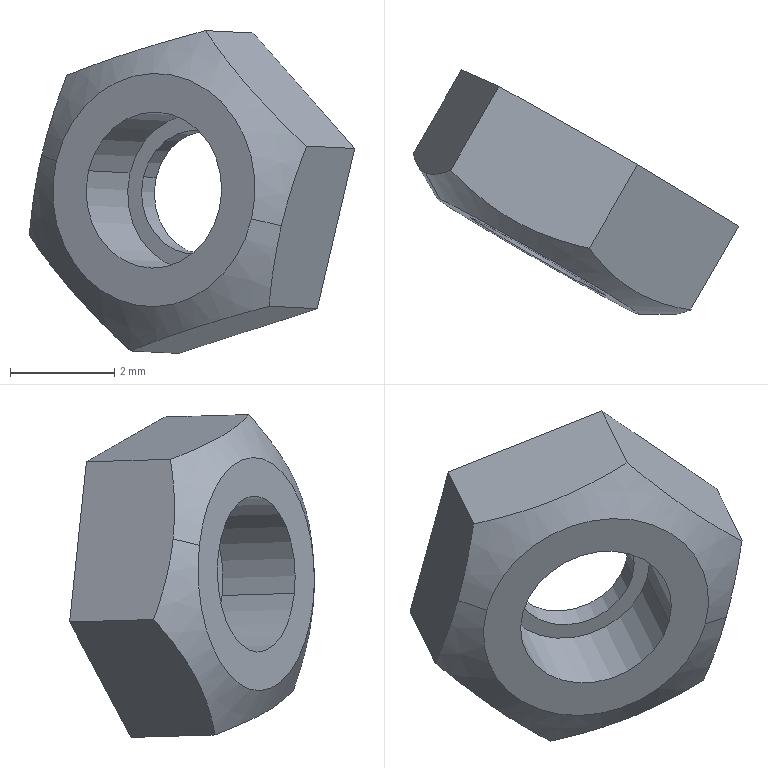Component | SolidWorks | KKSwitch-0710z0-123-1_CBTN3-0710z0-123-11 | 1 solid | 17 faces | box 6.25 x 4.7 x 6.2 mm | volume 45 mm3 | plane 9 | cylinder 4 | cone 4 | commonest cylinder face diameters 3 x2 2.386 x2
STEP:
#1=COLOUR_RGB('',0.7922,0.8196,0.9333);
#2=FILL_AREA_STYLE_COLOUR('',#1);
#3=FILL_AREA_STYLE('',(#2));
#4=SURFACE_STYLE_FILL_AREA(#3);
#5=SURFACE_SIDE_STYLE('',(#4));
#6=SURFACE_STYLE_USAGE(.BOTH.,#5);
#7=PRESENTATION_STYLE_ASSIGNMENT((#6));
#8=CARTESIAN_POINT('',(2.602,-0.2727,9.583));
#9=VERTEX_POINT('',#8);
#10=CARTESIAN_POINT('',(2.503,-0.2151,9.612));
#11=VERTEX_POINT('',#10);
#12=CARTESIAN_POINT('',(2.553,-0.2439,9.598));
#13=DIRECTION('',(-0.4977,-0.867,0.02519));
#14=DIRECTION('',(-0.8373,0.4878,0.2469));
#15=AXIS2_PLACEMENT_3D('',#12,#13,#14);
#16=CIRCLE('',#15,0.05906);
#17=EDGE_CURVE('',#9,#11,#16,.T.);
#18=ORIENTED_EDGE('',*,*,#17,.F.);
#19=CARTESIAN_POINT('',(2.571,-0.3273,9.585));
#20=VERTEX_POINT('',#19);
#21=CARTESIAN_POINT('',(2.54,-0.382,9.586));
#22=DIRECTION('',(-0.4977,-0.867,0.02519));
#23=VECTOR('',#22,39.37);
#24=LINE('',#21,#23);
#25=EDGE_CURVE('',#9,#20,#24,.T.);
#26=ORIENTED_EDGE('',*,*,#25,.T.);
#27=CARTESIAN_POINT('',(2.472,-0.2697,9.614));
#28=VERTEX_POINT('',#27);
#29=CARTESIAN_POINT('',(2.522,-0.2985,9.599));
#30=DIRECTION('',(-0.4977,-0.867,0.02519));
#31=DIRECTION('',(-0.8373,0.4878,0.2469));
#32=AXIS2_PLACEMENT_3D('',#29,#30,#31);
#33=CIRCLE('',#32,0.05906);
#34=EDGE_CURVE('',#20,#28,#33,.T.);
#35=ORIENTED_EDGE('',*,*,#34,.T.);
#36=CARTESIAN_POINT('',(2.441,-0.3243,9.615));
#37=DIRECTION('',(-0.4977,-0.867,0.02519));
#38=VECTOR('',#37,39.37);
#39=LINE('',#36,#38);
#40=EDGE_CURVE('',#11,#28,#39,.T.);
#41=ORIENTED_EDGE('',*,*,#40,.F.);
#42=EDGE_LOOP('',(#18,#26,#35,#41));
#43=FACE_OUTER_BOUND('',#42,.T.);
#44=CARTESIAN_POINT('',(2.49,-0.3531,9.601));
#45=DIRECTION('',(-0.4977,-0.867,0.02519));
#46=DIRECTION('',(-0.8373,0.4878,0.2469));
#47=AXIS2_PLACEMENT_3D('',#44,#45,#46);
#48=CYLINDRICAL_SURFACE('',#47,0.05906);
#49=ADVANCED_FACE('',(#43),#48,.F.);
#50=CARTESIAN_POINT('',(2.523,-0.2042,9.609));
#51=VERTEX_POINT('',#50);
#52=CARTESIAN_POINT('',(2.602,-0.25,9.586));
#53=VERTEX_POINT('',#52);
#54=CARTESIAN_POINT('',(2.563,-0.2271,9.597));
#55=DIRECTION('',(0.4977,0.867,-0.02519));
#56=DIRECTION('',(-0.2264,0.1018,-0.9687));
#57=AXIS2_PLACEMENT_3D('',#54,#55,#56);
#58=CIRCLE('',#57,0.04696);
#59=EDGE_CURVE('',#51,#53,#58,.T.);
#60=ORIENTED_EDGE('',*,*,#59,.F.);
#61=CARTESIAN_POINT('',(2.519,-0.1878,9.611));
#62=VERTEX_POINT('',#61);
#63=CARTESIAN_POINT('',(2.519,-0.1878,9.611));
#64=DIRECTION('',(-0.2401,0.958,0.1568));
#65=VECTOR('',#64,39.37);
#66=LINE('',#63,#65);
#67=EDGE_CURVE('',#51,#62,#66,.T.);
#68=ORIENTED_EDGE('',*,*,#67,.T.);
#69=CARTESIAN_POINT('',(2.618,-0.2454,9.582));
#70=VERTEX_POINT('',#69);
#71=CARTESIAN_POINT('',(2.569,-0.2166,9.597));
#72=DIRECTION('',(-0.4977,-0.867,0.02519));
#73=DIRECTION('',(0.8373,-0.4878,-0.2469));
#74=AXIS2_PLACEMENT_3D('',#71,#72,#73);
#75=CIRCLE('',#74,0.05906);
#76=EDGE_CURVE('',#70,#62,#75,.T.);
#77=ORIENTED_EDGE('',*,*,#76,.F.);
#78=CARTESIAN_POINT('',(2.618,-0.2454,9.582));
#79=DIRECTION('',(0.944,0.2681,-0.1924));
#80=VECTOR('',#79,39.37);
#81=LINE('',#78,#80);
#82=EDGE_CURVE('',#53,#70,#81,.T.);
#83=ORIENTED_EDGE('',*,*,#82,.F.);
#84=EDGE_LOOP('',(#60,#68,#77,#83));
#85=FACE_OUTER_BOUND('',#84,.T.);
#86=CARTESIAN_POINT('',(2.569,-0.2166,9.597));
#87=DIRECTION('',(0.4977,0.867,-0.02519));
#88=DIRECTION('',(0.8373,-0.4878,-0.2469));
#89=AXIS2_PLACEMENT_3D('',#86,#87,#88);
#90=CONICAL_SURFACE('',#89,0.05906,0.7854);
#91=ADVANCED_FACE('',(#85),#90,.F.);
#92=CARTESIAN_POINT('',(2.595,-0.3416,9.577));
#93=VERTEX_POINT('',#92);
#94=CARTESIAN_POINT('',(2.448,-0.2555,9.621));
#95=VERTEX_POINT('',#94);
#96=CARTESIAN_POINT('',(2.522,-0.2985,9.599));
#97=DIRECTION('',(0.4977,0.867,-0.02519));
#98=DIRECTION('',(0.8373,-0.4878,-0.2469));
#99=AXIS2_PLACEMENT_3D('',#96,#97,#98);
#100=CIRCLE('',#99,0.08819);
#101=EDGE_CURVE('',#93,#95,#100,.T.);
#102=ORIENTED_EDGE('',*,*,#101,.T.);
#103=CARTESIAN_POINT('',(2.437,-0.2357,9.626));
#104=VERTEX_POINT('',#103);
#105=CARTESIAN_POINT('',(2.427,-0.2189,9.63));
#106=DIRECTION('',(-0.4762,0.856,0.2013));
#107=VECTOR('',#106,39.37);
#108=LINE('',#105,#107);
#109=EDGE_CURVE('',#95,#104,#108,.T.);
#110=ORIENTED_EDGE('',*,*,#109,.T.);
#111=CARTESIAN_POINT('',(2.427,-0.2209,9.565));
#112=VERTEX_POINT('',#111);
#113=CARTESIAN_POINT('',(2.437,-0.2357,9.626));
#114=CARTESIAN_POINT('',(2.434,-0.2346,9.615));
#115=CARTESIAN_POINT('',(2.432,-0.2327,9.605));
#116=CARTESIAN_POINT('',(2.429,-0.2277,9.585));
#117=CARTESIAN_POINT('',(2.428,-0.2245,9.575));
#118=CARTESIAN_POINT('',(2.427,-0.2209,9.565));
#119=B_SPLINE_CURVE_WITH_KNOTS('',3,(#113,#114,#115,#116,#117,#118),.UNSPECIFIED.,.F.,.F.,(4,2,4),(0.001607,0.002407,0.003207),.UNSPECIFIED.);
#120=EDGE_CURVE('',#104,#112,#119,.T.);
#121=ORIENTED_EDGE('',*,*,#120,.T.);
#122=CARTESIAN_POINT('',(2.504,-0.2674,9.478));
#123=VERTEX_POINT('',#122);
#124=CARTESIAN_POINT('',(2.427,-0.2209,9.565));
#125=CARTESIAN_POINT('',(2.437,-0.2336,9.551));
#126=CARTESIAN_POINT('',(2.448,-0.2446,9.536));
#127=CARTESIAN_POINT('',(2.467,-0.2564,9.514));
#128=CARTESIAN_POINT('',(2.474,-0.2596,9.507));
#129=CARTESIAN_POINT('',(2.489,-0.2644,9.492));
#130=CARTESIAN_POINT('',(2.496,-0.2661,9.485));
#131=CARTESIAN_POINT('',(2.504,-0.2674,9.478));
#132=B_SPLINE_CURVE_WITH_KNOTS('',3,(#124,#125,#126,#127,#128,#129,#130,#131),.UNSPECIFIED.,.F.,.F.,(4,2,2,4),(0.,0.001604,0.002405,0.003207),.UNSPECIFIED.);
#133=EDGE_CURVE('',#112,#123,#132,.T.);
#134=ORIENTED_EDGE('',*,*,#133,.T.);
#135=CARTESIAN_POINT('',(2.609,-0.3266,9.511));
#136=VERTEX_POINT('',#135);
#137=CARTESIAN_POINT('',(2.504,-0.2674,9.478));
#138=CARTESIAN_POINT('',(2.518,-0.2821,9.483));
#139=CARTESIAN_POINT('',(2.534,-0.2952,9.489));
#140=CARTESIAN_POINT('',(2.56,-0.3103,9.498));
#141=CARTESIAN_POINT('',(2.57,-0.3146,9.5));
#142=CARTESIAN_POINT('',(2.589,-0.3215,9.506));
#143=CARTESIAN_POINT('',(2.599,-0.3243,9.509));
#144=CARTESIAN_POINT('',(2.609,-0.3266,9.511));
#145=B_SPLINE_CURVE_WITH_KNOTS('',3,(#137,#138,#139,#140,#141,#142,#143,#144),.UNSPECIFIED.,.F.,.F.,(4,2,2,4),(0.,0.001604,0.002405,0.003207),.UNSPECIFIED.);
#146=EDGE_CURVE('',#123,#136,#145,.T.);
#147=ORIENTED_EDGE('',*,*,#146,.T.);
#148=CARTESIAN_POINT('',(2.618,-0.3413,9.572));
#149=VERTEX_POINT('',#148);
#150=CARTESIAN_POINT('',(2.609,-0.3266,9.511));
#151=CARTESIAN_POINT('',(2.61,-0.3338,9.531));
#152=CARTESIAN_POINT('',(2.613,-0.3391,9.552));
#153=CARTESIAN_POINT('',(2.618,-0.3413,9.572));
#154=B_SPLINE_CURVE_WITH_KNOTS('',3,(#150,#151,#152,#153),.UNSPECIFIED.,.F.,.F.,(4,4),(0.,0.001607),.UNSPECIFIED.);
#155=EDGE_CURVE('',#136,#149,#154,.T.);
#156=ORIENTED_EDGE('',*,*,#155,.T.);
#157=CARTESIAN_POINT('',(2.637,-0.3411,9.568));
#158=DIRECTION('',(0.974,0.01101,-0.2265));
#159=VECTOR('',#158,39.37);
#160=LINE('',#157,#159);
#161=EDGE_CURVE('',#93,#149,#160,.T.);
#162=ORIENTED_EDGE('',*,*,#161,.F.);
#163=EDGE_LOOP('',(#102,#110,#121,#134,#147,#156,#162));
#164=FACE_OUTER_BOUND('',#163,.T.);
#165=CARTESIAN_POINT('',(2.532,-0.28,9.599));
#166=DIRECTION('',(0.4977,0.867,-0.02519));
#167=DIRECTION('',(0.8373,-0.4878,-0.2469));
#168=AXIS2_PLACEMENT_3D('',#165,#166,#167);
#169=CONICAL_SURFACE('',#168,0.1252,1.047);
#170=ADVANCED_FACE('',(#164),#169,.T.);
#171=CARTESIAN_POINT('',(2.514,-0.221,9.609));
#172=VERTEX_POINT('',#171);
#173=CARTESIAN_POINT('',(2.592,-0.2668,9.586));
#174=VERTEX_POINT('',#173);
#175=CARTESIAN_POINT('',(2.553,-0.2439,9.598));
#176=DIRECTION('',(0.4977,0.867,-0.02519));
#177=DIRECTION('',(-0.8373,0.4878,0.2469));
#178=AXIS2_PLACEMENT_3D('',#175,#176,#177);
#179=CIRCLE('',#178,0.04696);
#180=EDGE_CURVE('',#172,#174,#179,.T.);
#181=ORIENTED_EDGE('',*,*,#180,.F.);
#182=CARTESIAN_POINT('',(2.506,-0.2347,9.61));
#183=DIRECTION('',(0.4977,0.867,-0.02519));
#184=VECTOR('',#183,39.37);
#185=LINE('',#182,#184);
#186=EDGE_CURVE('',#172,#51,#185,.T.);
#187=ORIENTED_EDGE('',*,*,#186,.T.);
#188=ORIENTED_EDGE('',*,*,#59,.T.);
#189=CARTESIAN_POINT('',(2.584,-0.2805,9.586));
#190=DIRECTION('',(0.4977,0.867,-0.02519));
#191=VECTOR('',#190,39.37);
#192=LINE('',#189,#191);
#193=EDGE_CURVE('',#174,#53,#192,.T.);
#194=ORIENTED_EDGE('',*,*,#193,.F.);
#195=EDGE_LOOP('',(#181,#187,#188,#194));
#196=FACE_OUTER_BOUND('',#195,.T.);
#197=CARTESIAN_POINT('',(2.545,-0.2576,9.598));
#198=DIRECTION('',(0.4977,0.867,-0.02519));
#199=DIRECTION('',(0.8373,-0.4878,-0.2469));
#200=AXIS2_PLACEMENT_3D('',#197,#198,#199);
#201=CYLINDRICAL_SURFACE('',#200,0.04696);
#202=ADVANCED_FACE('',(#196),#201,.F.);
#203=ORIENTED_EDGE('',*,*,#186,.F.);
#204=CARTESIAN_POINT('',(2.553,-0.2439,9.598));
#205=DIRECTION('',(0.4977,0.867,-0.02519));
#206=DIRECTION('',(-0.8373,0.4878,0.2469));
#207=AXIS2_PLACEMENT_3D('',#204,#205,#206);
#208=CIRCLE('',#207,0.04696);
#209=EDGE_CURVE('',#174,#172,#208,.T.);
#210=ORIENTED_EDGE('',*,*,#209,.F.);
#211=ORIENTED_EDGE('',*,*,#193,.T.);
#212=CARTESIAN_POINT('',(2.563,-0.2271,9.597));
#213=DIRECTION('',(0.4977,0.867,-0.02519));
#214=DIRECTION('',(-0.2264,0.1018,-0.9687));
#215=AXIS2_PLACEMENT_3D('',#212,#213,#214);
#216=CIRCLE('',#215,0.04696);
#217=EDGE_CURVE('',#53,#51,#216,.T.);
#218=ORIENTED_EDGE('',*,*,#217,.T.);
#219=EDGE_LOOP('',(#203,#210,#211,#218));
#220=FACE_OUTER_BOUND('',#219,.T.);
#221=CARTESIAN_POINT('',(2.545,-0.2576,9.598));
#222=DIRECTION('',(0.4977,0.867,-0.02519));
#223=DIRECTION('',(0.8373,-0.4878,-0.2469));
#224=AXIS2_PLACEMENT_3D('',#221,#222,#223);
#225=CYLINDRICAL_SURFACE('',#224,0.04696);
#226=ADVANCED_FACE('',(#220),#225,.F.);
#227=ORIENTED_EDGE('',*,*,#76,.T.);
#228=CARTESIAN_POINT('',(2.569,-0.2166,9.597));
#229=DIRECTION('',(-0.4977,-0.867,0.02519));
#230=DIRECTION('',(0.8373,-0.4878,-0.2469));
#231=AXIS2_PLACEMENT_3D('',#228,#229,#230);
#232=CIRCLE('',#231,0.05906);
#233=EDGE_CURVE('',#62,#70,#232,.T.);
#234=ORIENTED_EDGE('',*,*,#233,.T.);
#235=EDGE_LOOP('',(#227,#234));
#236=FACE_BOUND('',#235,.T.);
#237=CARTESIAN_POINT('',(2.597,-0.2293,9.718));
#238=VERTEX_POINT('',#237);
#239=CARTESIAN_POINT('',(2.673,-0.2758,9.631));
#240=VERTEX_POINT('',#239);
#241=CARTESIAN_POINT('',(2.597,-0.2293,9.718));
#242=DIRECTION('',(0.6119,-0.3716,-0.6982));
#243=VECTOR('',#242,39.37);
#244=LINE('',#241,#243);
#245=EDGE_CURVE('',#238,#240,#244,.T.);
#246=ORIENTED_EDGE('',*,*,#245,.T.);
#247=CARTESIAN_POINT('',(2.645,-0.2631,9.51));
#248=VERTEX_POINT('',#247);
#249=CARTESIAN_POINT('',(2.644,-0.2624,9.503));
#250=DIRECTION('',(-0.2264,0.1018,-0.9687));
#251=VECTOR('',#250,39.37);
#252=LINE('',#249,#251);
#253=EDGE_CURVE('',#240,#248,#252,.T.);
#254=ORIENTED_EDGE('',*,*,#253,.T.);
#255=CARTESIAN_POINT('',(2.54,-0.2039,9.476));
#256=VERTEX_POINT('',#255);
#257=CARTESIAN_POINT('',(2.645,-0.2631,9.51));
#258=DIRECTION('',(-0.8383,0.4734,-0.2705));
#259=VECTOR('',#258,39.37);
#260=LINE('',#257,#259);
#261=EDGE_CURVE('',#248,#256,#260,.T.);
#262=ORIENTED_EDGE('',*,*,#261,.T.);
#263=CARTESIAN_POINT('',(2.464,-0.1574,9.563));
#264=VERTEX_POINT('',#263);
#265=CARTESIAN_POINT('',(2.54,-0.2039,9.476));
#266=DIRECTION('',(-0.6119,0.3716,0.6982));
#267=VECTOR('',#266,39.37);
#268=LINE('',#265,#267);
#269=EDGE_CURVE('',#256,#264,#268,.T.);
#270=ORIENTED_EDGE('',*,*,#269,.T.);
#271=CARTESIAN_POINT('',(2.492,-0.1702,9.684));
#272=VERTEX_POINT('',#271);
#273=CARTESIAN_POINT('',(2.462,-0.1567,9.556));
#274=DIRECTION('',(0.2264,-0.1018,0.9687));
#275=VECTOR('',#274,39.37);
#276=LINE('',#273,#275);
#277=EDGE_CURVE('',#264,#272,#276,.T.);
#278=ORIENTED_EDGE('',*,*,#277,.T.);
#279=CARTESIAN_POINT('',(2.492,-0.1702,9.684));
#280=DIRECTION('',(0.8383,-0.4734,0.2705));
#281=VECTOR('',#280,39.37);
#282=LINE('',#279,#281);
#283=EDGE_CURVE('',#272,#238,#282,.T.);
#284=ORIENTED_EDGE('',*,*,#283,.T.);
#285=EDGE_LOOP('',(#246,#254,#262,#270,#278,#284));
#286=FACE_OUTER_BOUND('',#285,.T.);
#287=CARTESIAN_POINT('',(2.553,-0.2096,9.53));
#288=DIRECTION('',(0.4977,0.867,-0.02519));
#289=DIRECTION('',(0.8373,-0.4878,-0.2469));
#290=AXIS2_PLACEMENT_3D('',#287,#288,#289);
#291=PLANE('',#290);
#292=ADVANCED_FACE('',(#236,#286),#291,.T.);
#293=ORIENTED_EDGE('',*,*,#67,.F.);
#294=ORIENTED_EDGE('',*,*,#217,.F.);
#295=ORIENTED_EDGE('',*,*,#82,.T.);
#296=ORIENTED_EDGE('',*,*,#233,.F.);
#297=EDGE_LOOP('',(#293,#294,#295,#296));
#298=FACE_OUTER_BOUND('',#297,.T.);
#299=CARTESIAN_POINT('',(2.569,-0.2166,9.597));
#300=DIRECTION('',(0.4977,0.867,-0.02519));
#301=DIRECTION('',(0.8373,-0.4878,-0.2469));
#302=AXIS2_PLACEMENT_3D('',#299,#300,#301);
#303=CONICAL_SURFACE('',#302,0.05906,0.7854);
#304=ADVANCED_FACE('',(#298),#303,.F.);
#305=CARTESIAN_POINT('',(2.645,-0.2631,9.51));
#306=DIRECTION('',(-0.4977,-0.867,0.02519));
#307=VECTOR('',#306,39.37);
#308=LINE('',#305,#307);
#309=EDGE_CURVE('',#248,#136,#308,.T.);
#310=ORIENTED_EDGE('',*,*,#309,.F.);
#311=ORIENTED_EDGE('',*,*,#253,.F.);
#312=CARTESIAN_POINT('',(2.637,-0.3393,9.633));
#313=VERTEX_POINT('',#312);
#314=CARTESIAN_POINT('',(2.673,-0.2758,9.631));
#315=DIRECTION('',(0.4977,0.867,-0.02519));
#316=VECTOR('',#315,39.37);
#317=LINE('',#314,#316);
#318=EDGE_CURVE('',#313,#240,#317,.T.);
#319=ORIENTED_EDGE('',*,*,#318,.F.);
#320=CARTESIAN_POINT('',(2.618,-0.3413,9.572));
#321=CARTESIAN_POINT('',(2.62,-0.3424,9.582));
#322=CARTESIAN_POINT('',(2.623,-0.3427,9.593));
#323=CARTESIAN_POINT('',(2.63,-0.3419,9.613));
#324=CARTESIAN_POINT('',(2.633,-0.3408,9.623));
#325=CARTESIAN_POINT('',(2.637,-0.3393,9.633));
#326=B_SPLINE_CURVE_WITH_KNOTS('',3,(#320,#321,#322,#323,#324,#325),.UNSPECIFIED.,.F.,.F.,(4,2,4),(0.001607,0.002407,0.003207),.UNSPECIFIED.);
#327=EDGE_CURVE('',#149,#313,#326,.T.);
#328=ORIENTED_EDGE('',*,*,#327,.F.);
#329=ORIENTED_EDGE('',*,*,#155,.F.);
#330=EDGE_LOOP('',(#310,#311,#319,#328,#329));
#331=FACE_OUTER_BOUND('',#330,.T.);
#332=CARTESIAN_POINT('',(2.645,-0.2631,9.51));
#333=DIRECTION('',(-0.8373,0.4878,0.2469));
#334=DIRECTION('',(0.4977,0.867,-0.02519));
#335=AXIS2_PLACEMENT_3D('',#332,#333,#334);
#336=PLANE('',#335);
#337=ADVANCED_FACE('',(#331),#336,.F.);
#338=ORIENTED_EDGE('',*,*,#318,.T.);
#339=ORIENTED_EDGE('',*,*,#245,.F.);
#340=CARTESIAN_POINT('',(2.56,-0.2928,9.72));
#341=VERTEX_POINT('',#340);
#342=CARTESIAN_POINT('',(2.597,-0.2293,9.718));
#343=DIRECTION('',(0.4977,0.867,-0.02519));
#344=VECTOR('',#343,39.37);
#345=LINE('',#342,#344);
#346=EDGE_CURVE('',#341,#238,#345,.T.);
#347=ORIENTED_EDGE('',*,*,#346,.F.);
#348=CARTESIAN_POINT('',(2.637,-0.3393,9.633));
#349=CARTESIAN_POINT('',(2.622,-0.3368,9.647));
#350=CARTESIAN_POINT('',(2.607,-0.3324,9.661));
#351=CARTESIAN_POINT('',(2.587,-0.3205,9.684));
#352=CARTESIAN_POINT('',(2.581,-0.3158,9.691));
#353=CARTESIAN_POINT('',(2.57,-0.3051,9.706));
#354=CARTESIAN_POINT('',(2.565,-0.2992,9.713));
#355=CARTESIAN_POINT('',(2.56,-0.2928,9.72));
#356=B_SPLINE_CURVE_WITH_KNOTS('',3,(#348,#349,#350,#351,#352,#353,#354,#355),.UNSPECIFIED.,.F.,.F.,(4,2,2,4),(0.,0.001604,0.002405,0.003207),.UNSPECIFIED.);
#357=EDGE_CURVE('',#313,#341,#356,.T.);
#358=ORIENTED_EDGE('',*,*,#357,.F.);
#359=EDGE_LOOP('',(#338,#339,#347,#358));
#360=FACE_OUTER_BOUND('',#359,.T.);
#361=CARTESIAN_POINT('',(2.673,-0.2758,9.631));
#362=DIRECTION('',(-0.6147,0.3321,-0.7154));
#363=DIRECTION('',(-0.6119,0.3716,0.6982));
#364=AXIS2_PLACEMENT_3D('',#361,#362,#363);
#365=PLANE('',#364);
#366=ADVANCED_FACE('',(#360),#365,.F.);
#367=ORIENTED_EDGE('',*,*,#346,.T.);
#368=ORIENTED_EDGE('',*,*,#283,.F.);
#369=CARTESIAN_POINT('',(2.456,-0.2336,9.686));
#370=VERTEX_POINT('',#369);
#371=CARTESIAN_POINT('',(2.492,-0.1702,9.684));
#372=DIRECTION('',(0.4977,0.867,-0.02519));
#373=VECTOR('',#372,39.37);
#374=LINE('',#371,#373);
#375=EDGE_CURVE('',#370,#272,#374,.T.);
#376=ORIENTED_EDGE('',*,*,#375,.F.);
#377=CARTESIAN_POINT('',(2.56,-0.2928,9.72));
#378=CARTESIAN_POINT('',(2.54,-0.2883,9.714));
#379=CARTESIAN_POINT('',(2.521,-0.2817,9.709));
#380=CARTESIAN_POINT('',(2.494,-0.2667,9.7));
#381=CARTESIAN_POINT('',(2.486,-0.2608,9.697));
#382=CARTESIAN_POINT('',(2.47,-0.248,9.692));
#383=CARTESIAN_POINT('',(2.463,-0.241,9.689));
#384=CARTESIAN_POINT('',(2.456,-0.2336,9.686));
#385=B_SPLINE_CURVE_WITH_KNOTS('',3,(#377,#378,#379,#380,#381,#382,#383,#384),.UNSPECIFIED.,.F.,.F.,(4,2,2,4),(0.,0.001604,0.002405,0.003207),.UNSPECIFIED.);
#386=EDGE_CURVE('',#341,#370,#385,.T.);
#387=ORIENTED_EDGE('',*,*,#386,.F.);
#388=EDGE_LOOP('',(#367,#368,#376,#387));
#389=FACE_OUTER_BOUND('',#388,.T.);
#390=CARTESIAN_POINT('',(2.597,-0.2293,9.718));
#391=DIRECTION('',(0.2226,-0.1557,-0.9624));
#392=DIRECTION('',(-0.8383,0.4734,-0.2705));
#393=AXIS2_PLACEMENT_3D('',#390,#391,#392);
#394=PLANE('',#393);
#395=ADVANCED_FACE('',(#389),#394,.F.);
#396=ORIENTED_EDGE('',*,*,#375,.T.);
#397=ORIENTED_EDGE('',*,*,#277,.F.);
#398=CARTESIAN_POINT('',(2.464,-0.1574,9.563));
#399=DIRECTION('',(0.4977,0.867,-0.02519));
#400=VECTOR('',#399,39.37);
#401=LINE('',#398,#400);
#402=EDGE_CURVE('',#112,#264,#401,.T.);
#403=ORIENTED_EDGE('',*,*,#402,.F.);
#404=ORIENTED_EDGE('',*,*,#120,.F.);
#405=CARTESIAN_POINT('',(2.456,-0.2336,9.686));
#406=CARTESIAN_POINT('',(2.448,-0.2367,9.666));
#407=CARTESIAN_POINT('',(2.442,-0.2378,9.646));
#408=CARTESIAN_POINT('',(2.437,-0.2357,9.626));
#409=B_SPLINE_CURVE_WITH_KNOTS('',3,(#405,#406,#407,#408),.UNSPECIFIED.,.F.,.F.,(4,4),(0.,0.001607),.UNSPECIFIED.);
#410=EDGE_CURVE('',#370,#104,#409,.T.);
#411=ORIENTED_EDGE('',*,*,#410,.F.);
#412=EDGE_LOOP('',(#396,#397,#403,#404,#411));
#413=FACE_OUTER_BOUND('',#412,.T.);
#414=CARTESIAN_POINT('',(2.492,-0.1702,9.684));
#415=DIRECTION('',(0.8373,-0.4878,-0.2469));
#416=DIRECTION('',(-0.4977,-0.867,0.02519));
#417=AXIS2_PLACEMENT_3D('',#414,#415,#416);
#418=PLANE('',#417);
#419=ADVANCED_FACE('',(#413),#418,.F.);
#420=ORIENTED_EDGE('',*,*,#402,.T.);
#421=ORIENTED_EDGE('',*,*,#269,.F.);
#422=CARTESIAN_POINT('',(2.54,-0.2039,9.476));
#423=DIRECTION('',(0.4977,0.867,-0.02519));
#424=VECTOR('',#423,39.37);
#425=LINE('',#422,#424);
#426=EDGE_CURVE('',#123,#256,#425,.T.);
#427=ORIENTED_EDGE('',*,*,#426,.F.);
#428=ORIENTED_EDGE('',*,*,#133,.F.);
#429=EDGE_LOOP('',(#420,#421,#427,#428));
#430=FACE_OUTER_BOUND('',#429,.T.);
#431=CARTESIAN_POINT('',(2.464,-0.1574,9.563));
#432=DIRECTION('',(0.6147,-0.3321,0.7154));
#433=DIRECTION('',(0.6119,-0.3716,-0.6982));
#434=AXIS2_PLACEMENT_3D('',#431,#432,#433);
#435=PLANE('',#434);
#436=ADVANCED_FACE('',(#430),#435,.F.);
#437=ORIENTED_EDGE('',*,*,#426,.T.);
#438=ORIENTED_EDGE('',*,*,#261,.F.);
#439=ORIENTED_EDGE('',*,*,#309,.T.);
#440=ORIENTED_EDGE('',*,*,#146,.F.);
#441=EDGE_LOOP('',(#437,#438,#439,#440));
#442=FACE_OUTER_BOUND('',#441,.T.);
#443=CARTESIAN_POINT('',(2.54,-0.2039,9.476));
#444=DIRECTION('',(-0.2226,0.1557,0.9624));
#445=DIRECTION('',(0.8383,-0.4734,0.2705));
#446=AXIS2_PLACEMENT_3D('',#443,#444,#445);
#447=PLANE('',#446);
#448=ADVANCED_FACE('',(#442),#447,.F.);
#449=ORIENTED_EDGE('',*,*,#109,.F.);
#450=CARTESIAN_POINT('',(2.522,-0.2985,9.599));
#451=DIRECTION('',(0.4977,0.867,-0.02519));
#452=DIRECTION('',(0.8373,-0.4878,-0.2469));
#453=AXIS2_PLACEMENT_3D('',#450,#451,#452);
#454=CIRCLE('',#453,0.08819);
#455=EDGE_CURVE('',#95,#93,#454,.T.);
#456=ORIENTED_EDGE('',*,*,#455,.T.);
#457=ORIENTED_EDGE('',*,*,#161,.T.);
#458=ORIENTED_EDGE('',*,*,#327,.T.);
#459=ORIENTED_EDGE('',*,*,#357,.T.);
#460=ORIENTED_EDGE('',*,*,#386,.T.);
#461=ORIENTED_EDGE('',*,*,#410,.T.);
#462=EDGE_LOOP('',(#449,#456,#457,#458,#459,#460,#461));
#463=FACE_OUTER_BOUND('',#462,.T.);
#464=CARTESIAN_POINT('',(2.532,-0.28,9.599));
#465=DIRECTION('',(0.4977,0.867,-0.02519));
#466=DIRECTION('',(0.8373,-0.4878,-0.2469));
#467=AXIS2_PLACEMENT_3D('',#464,#465,#466);
#468=CONICAL_SURFACE('',#467,0.1252,1.047);
#469=ADVANCED_FACE('',(#463),#468,.T.);
#470=ORIENTED_EDGE('',*,*,#101,.F.);
#471=ORIENTED_EDGE('',*,*,#455,.F.);
#472=EDGE_LOOP('',(#470,#471));
#473=FACE_OUTER_BOUND('',#472,.T.);
#474=CARTESIAN_POINT('',(2.522,-0.2985,9.599));
#475=DIRECTION('',(-0.4977,-0.867,0.02519));
#476=DIRECTION('',(-0.8373,0.4878,0.2469));
#477=AXIS2_PLACEMENT_3D('',#474,#475,#476);
#478=CIRCLE('',#477,0.05906);
#479=EDGE_CURVE('',#28,#20,#478,.T.);
#480=ORIENTED_EDGE('',*,*,#479,.F.);
#481=ORIENTED_EDGE('',*,*,#34,.F.);
#482=EDGE_LOOP('',(#480,#481));
#483=FACE_BOUND('',#482,.T.);
#484=CARTESIAN_POINT('',(2.512,-0.294,9.557));
#485=DIRECTION('',(-0.4977,-0.867,0.02519));
#486=DIRECTION('',(-0.8373,0.4878,0.2469));
#487=AXIS2_PLACEMENT_3D('',#484,#485,#486);
#488=PLANE('',#487);
#489=ADVANCED_FACE('',(#473,#483),#488,.T.);
#490=ORIENTED_EDGE('',*,*,#25,.F.);
#491=CARTESIAN_POINT('',(2.553,-0.2439,9.598));
#492=DIRECTION('',(-0.4977,-0.867,0.02519));
#493=DIRECTION('',(-0.8373,0.4878,0.2469));
#494=AXIS2_PLACEMENT_3D('',#491,#492,#493);
#495=CIRCLE('',#494,0.05906);
#496=EDGE_CURVE('',#11,#9,#495,.T.);
#497=ORIENTED_EDGE('',*,*,#496,.F.);
#498=ORIENTED_EDGE('',*,*,#40,.T.);
#499=ORIENTED_EDGE('',*,*,#479,.T.);
#500=EDGE_LOOP('',(#490,#497,#498,#499));
#501=FACE_OUTER_BOUND('',#500,.T.);
#502=CARTESIAN_POINT('',(2.49,-0.3531,9.601));
#503=DIRECTION('',(-0.4977,-0.867,0.02519));
#504=DIRECTION('',(-0.8373,0.4878,0.2469));
#505=AXIS2_PLACEMENT_3D('',#502,#503,#504);
#506=CYLINDRICAL_SURFACE('',#505,0.05906);
#507=ADVANCED_FACE('',(#501),#506,.F.);
#508=ORIENTED_EDGE('',*,*,#496,.T.);
#509=ORIENTED_EDGE('',*,*,#17,.T.);
#510=EDGE_LOOP('',(#508,#509));
#511=FACE_OUTER_BOUND('',#510,.T.);
#512=ORIENTED_EDGE('',*,*,#209,.T.);
#513=ORIENTED_EDGE('',*,*,#180,.T.);
#514=EDGE_LOOP('',(#512,#513));
#515=FACE_BOUND('',#514,.T.);
#516=CARTESIAN_POINT('',(2.553,-0.2439,9.598));
#517=DIRECTION('',(-0.4977,-0.867,0.02519));
#518=DIRECTION('',(-0.8373,0.4878,0.2469));
#519=AXIS2_PLACEMENT_3D('',#516,#517,#518);
#520=PLANE('',#519);
#521=ADVANCED_FACE('',(#511,#515),#520,.T.);
#522=CLOSED_SHELL('',(#49,#91,#170,#202,#226,#292,#304,#337,#366,#395,#419,#436,#448,#469,#489,#507,#521));
#523=MANIFOLD_SOLID_BREP('',#522);
#524=STYLED_ITEM('',(#7),#523);
#525=(LENGTH_UNIT()NAMED_UNIT(*)SI_UNIT($,.METRE.));
#526=LENGTH_MEASURE_WITH_UNIT(LENGTH_MEASURE(0.0254),#525);
#527=DIMENSIONAL_EXPONENTS(1.,0.,0.,0.,0.,0.,0.);
#528=(CONVERSION_BASED_UNIT('',#526)LENGTH_UNIT()NAMED_UNIT(#527));
#529=UNCERTAINTY_MEASURE_WITH_UNIT(LENGTH_MEASURE(0.00001),#528,'','');
#530=(NAMED_UNIT(*)PLANE_ANGLE_UNIT()SI_UNIT($,.RADIAN.));
#531=(NAMED_UNIT(*)SI_UNIT($,.STERADIAN.)SOLID_ANGLE_UNIT());
#532=(GEOMETRIC_REPRESENTATION_CONTEXT(3)GLOBAL_UNCERTAINTY_ASSIGNED_CONTEXT((#529))GLOBAL_UNIT_ASSIGNED_CONTEXT((#528,#530,#531))REPRESENTATION_CONTEXT('',''));
#533=MECHANICAL_DESIGN_GEOMETRIC_PRESENTATION_REPRESENTATION('',(#524),#532);
#534=PRESENTATION_LAYER_ASSIGNMENT('','',(#524));
#535=CARTESIAN_POINT('',(0.,0.,0.));
#536=DIRECTION('',(0.,0.,1.));
#537=DIRECTION('',(1.,0.,0.));
#538=AXIS2_PLACEMENT_3D('',#535,#536,#537);
#539=(LENGTH_UNIT()NAMED_UNIT(*)SI_UNIT($,.METRE.));
#540=LENGTH_MEASURE_WITH_UNIT(LENGTH_MEASURE(0.0254),#539);
#541=DIMENSIONAL_EXPONENTS(1.,0.,0.,0.,0.,0.,0.);
#542=(CONVERSION_BASED_UNIT('',#540)LENGTH_UNIT()NAMED_UNIT(#541));
#543=UNCERTAINTY_MEASURE_WITH_UNIT(LENGTH_MEASURE(0.00001),#542,'','');
#544=(NAMED_UNIT(*)PLANE_ANGLE_UNIT()SI_UNIT($,.RADIAN.));
#545=(NAMED_UNIT(*)SI_UNIT($,.STERADIAN.)SOLID_ANGLE_UNIT());
#546=(GEOMETRIC_REPRESENTATION_CONTEXT(3)GLOBAL_UNCERTAINTY_ASSIGNED_CONTEXT((#543))GLOBAL_UNIT_ASSIGNED_CONTEXT((#542,#544,#545))REPRESENTATION_CONTEXT('',''));
#547=ADVANCED_BREP_SHAPE_REPRESENTATION('',(#523,#538),#546);